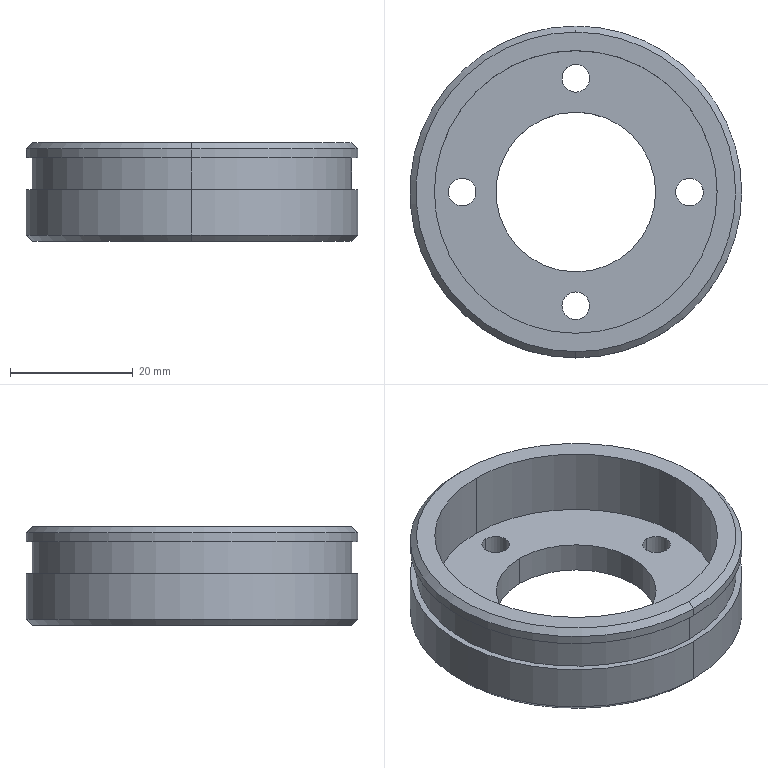CAM job | Mastercam | mm | 1 operations | part box 54 x 54 x 16
1. Drill/Counterbore | 7 - 4 倒角刀